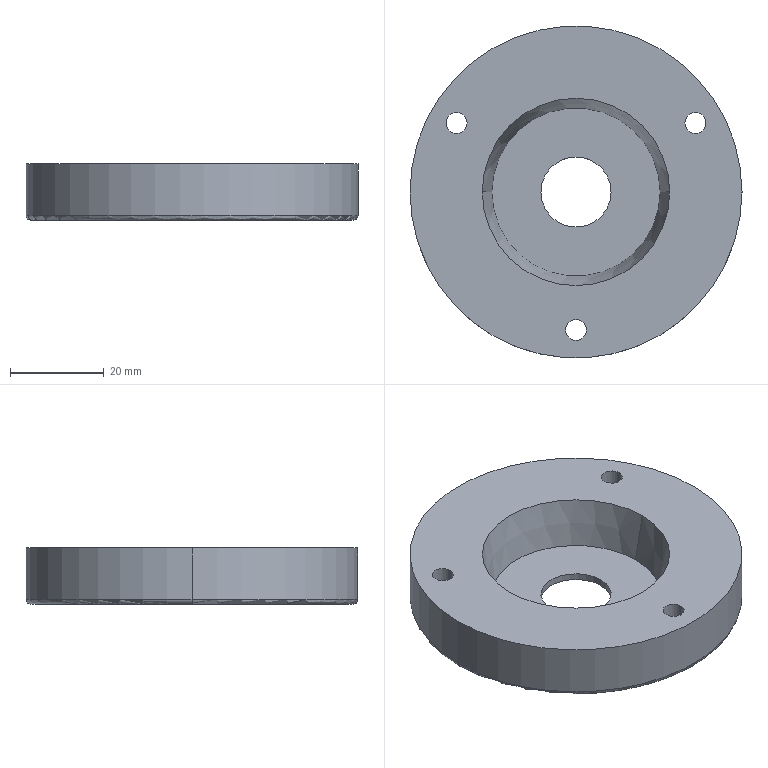Component | SolidWorks | SealingCover-2 | 1 solid | 26 faces | box 71 x 71 x 12 mm | volume 34206 mm3 | cylinder 16 | plane 6 | torus 2 | cone 2 | commonest cylinder face diameters 8 x6 4.5 x6 15 x2 71 x2
build123d program:
from build123d import *

# Parameters (mm, degrees)
SKETCH1_R                                            = 35.5
BOSS_EXTRUDE1_DEPTH                                  = 12
HOLE_SIZE_ACCORDING_TO_HEXAGON_SOCKET_HE_D           = 4.5
HOLE_SIZE_ACCORDING_TO_HEXAGON_SOCKET_HE_CBORE_D     = 8
HOLE_SIZE_ACCORDING_TO_HEXAGON_SOCKET_HE_CBORE_DEPTH = 4.6
CIRPATTERN1_COUNT                                    = 3
FILLET1_R                                            = 1


with BuildPart() as part:
    # Sketch1 → Boss-Extrude1 (new body)
    with BuildSketch(Plane.XY):
        Circle(SKETCH1_R)
    extrude(amount=-BOSS_EXTRUDE1_DEPTH)

    # Sketch2 → Cut-Revolve1 (revolve, cut)
    with BuildSketch(Plane(origin=(0, 0, 0), x_dir=(1, 0, 0), z_dir=(0, 1, 0)), mode=Mode.PRIVATE) as cut_revolve1_sk:
        Polygon((-18, 1.5), (-7.5, 1.5), (-7.5, 0), (0, 0), (0, 12), (-20.041, 12), align=None)
    revolve(cut_revolve1_sk.sketch.rotate(Axis((0, 0, 0), (0, 0, -1)), 180), axis=Axis((0, 0, 0), (0, 0, -1)), mode=Mode.SUBTRACT)

    # Hole Size_According to_Hexagon Socket He (through all)
    with Locations(Plane.XY):
        with Locations((0, -29.5)):
            hole_size_according_to_hexagon_socket_he = CounterBoreHole(HOLE_SIZE_ACCORDING_TO_HEXAGON_SOCKET_HE_D / 2, HOLE_SIZE_ACCORDING_TO_HEXAGON_SOCKET_HE_CBORE_D / 2, HOLE_SIZE_ACCORDING_TO_HEXAGON_SOCKET_HE_CBORE_DEPTH)

    # CirPattern1: Hole Size_According to_Hexagon Socket He ×3 about axis
    cirpattern1_axis = Axis((0, 0, 0), (0, 0, 1))
    for i in range(1, CIRPATTERN1_COUNT):
        add(hole_size_according_to_hexagon_socket_he.rotate(cirpattern1_axis, i * 360 / CIRPATTERN1_COUNT), mode=Mode.SUBTRACT)

    # Fillet1
    fillet1_edges = [part.edges().sort_by_distance(p)[0] for p in [
        (-35.5, 0, 0),
    ]]
    fillet(fillet1_edges, radius=FILLET1_R)


solid = part.part

# Placed as in the assembly
solid = solid.moved(Location((32, 58.948, -59), (-180, 0, 180)))
STEP:
#1=COLOUR_RGB('',0.7922,0.8196,0.9333);
#2=FILL_AREA_STYLE_COLOUR('',#1);
#3=FILL_AREA_STYLE('',(#2));
#4=SURFACE_STYLE_FILL_AREA(#3);
#5=SURFACE_SIDE_STYLE('',(#4));
#6=SURFACE_STYLE_USAGE(.BOTH.,#5);
#7=PRESENTATION_STYLE_ASSIGNMENT((#6));
#8=CARTESIAN_POINT('',(2.657,2.321,-2.283));
#9=VERTEX_POINT('',#8);
#10=CARTESIAN_POINT('',(-0.1378,2.321,-2.283));
#11=VERTEX_POINT('',#10);
#12=CARTESIAN_POINT('',(1.26,2.321,-2.283));
#13=DIRECTION('',(0.,0.,1.));
#14=DIRECTION('',(-1.,-0.,0.));
#15=AXIS2_PLACEMENT_3D('',#12,#13,#14);
#16=CIRCLE('',#15,1.398);
#17=EDGE_CURVE('',#9,#11,#16,.T.);
#18=ORIENTED_EDGE('',*,*,#17,.F.);
#19=CARTESIAN_POINT('',(2.618,2.321,-2.323));
#20=VERTEX_POINT('',#19);
#21=CARTESIAN_POINT('',(2.618,2.321,-2.283));
#22=DIRECTION('',(-0.,1.,-0.));
#23=DIRECTION('',(-1.,0.,0.));
#24=AXIS2_PLACEMENT_3D('',#21,#22,#23);
#25=CIRCLE('',#24,0.03937);
#26=EDGE_CURVE('',#9,#20,#25,.T.);
#27=ORIENTED_EDGE('',*,*,#26,.T.);
#28=CARTESIAN_POINT('',(-0.09843,2.321,-2.323));
#29=VERTEX_POINT('',#28);
#30=CARTESIAN_POINT('',(1.26,2.321,-2.323));
#31=DIRECTION('',(-0.,-0.,-1.));
#32=DIRECTION('',(-1.,-0.,0.));
#33=AXIS2_PLACEMENT_3D('',#30,#31,#32);
#34=CIRCLE('',#33,1.358);
#35=EDGE_CURVE('',#29,#20,#34,.T.);
#36=ORIENTED_EDGE('',*,*,#35,.F.);
#37=CARTESIAN_POINT('',(-0.09843,2.321,-2.283));
#38=DIRECTION('',(0.,-1.,0.));
#39=DIRECTION('',(1.,0.,0.));
#40=AXIS2_PLACEMENT_3D('',#37,#38,#39);
#41=CIRCLE('',#40,0.03937);
#42=EDGE_CURVE('',#11,#29,#41,.T.);
#43=ORIENTED_EDGE('',*,*,#42,.F.);
#44=EDGE_LOOP('',(#18,#27,#36,#43));
#45=FACE_OUTER_BOUND('',#44,.T.);
#46=CARTESIAN_POINT('',(1.26,2.321,-2.283));
#47=DIRECTION('',(-0.,-0.,-1.));
#48=DIRECTION('',(-1.,-0.,0.));
#49=AXIS2_PLACEMENT_3D('',#46,#47,#48);
#50=TOROIDAL_SURFACE('',#49,1.358,0.03937);
#51=ADVANCED_FACE('',(#45),#50,.T.);
#52=CARTESIAN_POINT('',(0.4115,2.901,-2.142));
#53=VERTEX_POINT('',#52);
#54=CARTESIAN_POINT('',(0.09655,2.901,-2.142));
#55=VERTEX_POINT('',#54);
#56=CARTESIAN_POINT('',(0.254,2.901,-2.142));
#57=DIRECTION('',(-0.,-0.,-1.));
#58=DIRECTION('',(-1.,0.,0.));
#59=AXIS2_PLACEMENT_3D('',#56,#57,#58);
#60=CIRCLE('',#59,0.1575);
#61=EDGE_CURVE('',#53,#55,#60,.T.);
#62=ORIENTED_EDGE('',*,*,#61,.F.);
#63=CARTESIAN_POINT('',(0.4115,2.901,-2.323));
#64=VERTEX_POINT('',#63);
#65=CARTESIAN_POINT('',(0.4115,2.901,-2.323));
#66=DIRECTION('',(-0.,-0.,-1.));
#67=VECTOR('',#66,39.37);
#68=LINE('',#65,#67);
#69=EDGE_CURVE('',#53,#64,#68,.T.);
#70=ORIENTED_EDGE('',*,*,#69,.T.);
#71=CARTESIAN_POINT('',(0.09655,2.901,-2.323));
#72=VERTEX_POINT('',#71);
#73=CARTESIAN_POINT('',(0.254,2.901,-2.323));
#74=DIRECTION('',(-0.,-0.,-1.));
#75=DIRECTION('',(-1.,0.,0.));
#76=AXIS2_PLACEMENT_3D('',#73,#74,#75);
#77=CIRCLE('',#76,0.1575);
#78=EDGE_CURVE('',#64,#72,#77,.T.);
#79=ORIENTED_EDGE('',*,*,#78,.T.);
#80=CARTESIAN_POINT('',(0.09655,2.901,-2.323));
#81=DIRECTION('',(-0.,-0.,-1.));
#82=VECTOR('',#81,39.37);
#83=LINE('',#80,#82);
#84=EDGE_CURVE('',#55,#72,#83,.T.);
#85=ORIENTED_EDGE('',*,*,#84,.F.);
#86=EDGE_LOOP('',(#62,#70,#79,#85));
#87=FACE_OUTER_BOUND('',#86,.T.);
#88=CARTESIAN_POINT('',(0.254,2.901,-2.323));
#89=DIRECTION('',(-0.,-0.,-1.));
#90=DIRECTION('',(-1.,0.,0.));
#91=AXIS2_PLACEMENT_3D('',#88,#89,#90);
#92=CYLINDRICAL_SURFACE('',#91,0.1575);
#93=ADVANCED_FACE('',(#87),#92,.F.);
#94=CARTESIAN_POINT('',(0.3426,2.901,-1.85));
#95=VERTEX_POINT('',#94);
#96=CARTESIAN_POINT('',(0.1654,2.901,-1.85));
#97=VERTEX_POINT('',#96);
#98=CARTESIAN_POINT('',(0.254,2.901,-1.85));
#99=DIRECTION('',(-0.,-0.,-1.));
#100=DIRECTION('',(-1.,0.,0.));
#101=AXIS2_PLACEMENT_3D('',#98,#99,#100);
#102=CIRCLE('',#101,0.08858);
#103=EDGE_CURVE('',#95,#97,#102,.T.);
#104=ORIENTED_EDGE('',*,*,#103,.F.);
#105=CARTESIAN_POINT('',(0.3426,2.901,-2.142));
#106=VERTEX_POINT('',#105);
#107=CARTESIAN_POINT('',(0.3426,2.901,-2.323));
#108=DIRECTION('',(-0.,-0.,-1.));
#109=VECTOR('',#108,39.37);
#110=LINE('',#107,#109);
#111=EDGE_CURVE('',#95,#106,#110,.T.);
#112=ORIENTED_EDGE('',*,*,#111,.T.);
#113=CARTESIAN_POINT('',(0.1654,2.901,-2.142));
#114=VERTEX_POINT('',#113);
#115=CARTESIAN_POINT('',(0.254,2.901,-2.142));
#116=DIRECTION('',(-0.,-0.,-1.));
#117=DIRECTION('',(-1.,0.,0.));
#118=AXIS2_PLACEMENT_3D('',#115,#116,#117);
#119=CIRCLE('',#118,0.08858);
#120=EDGE_CURVE('',#106,#114,#119,.T.);
#121=ORIENTED_EDGE('',*,*,#120,.T.);
#122=CARTESIAN_POINT('',(0.1654,2.901,-2.323));
#123=DIRECTION('',(-0.,-0.,-1.));
#124=VECTOR('',#123,39.37);
#125=LINE('',#122,#124);
#126=EDGE_CURVE('',#97,#114,#125,.T.);
#127=ORIENTED_EDGE('',*,*,#126,.F.);
#128=EDGE_LOOP('',(#104,#112,#121,#127));
#129=FACE_OUTER_BOUND('',#128,.T.);
#130=CARTESIAN_POINT('',(0.254,2.901,-2.323));
#131=DIRECTION('',(-0.,-0.,-1.));
#132=DIRECTION('',(-1.,0.,0.));
#133=AXIS2_PLACEMENT_3D('',#130,#131,#132);
#134=CYLINDRICAL_SURFACE('',#133,0.08858);
#135=ADVANCED_FACE('',(#129),#134,.F.);
#136=CARTESIAN_POINT('',(2.423,2.901,-2.142));
#137=VERTEX_POINT('',#136);
#138=CARTESIAN_POINT('',(2.108,2.901,-2.142));
#139=VERTEX_POINT('',#138);
#140=CARTESIAN_POINT('',(2.266,2.901,-2.142));
#141=DIRECTION('',(-0.,-0.,-1.));
#142=DIRECTION('',(-1.,0.,0.));
#143=AXIS2_PLACEMENT_3D('',#140,#141,#142);
#144=CIRCLE('',#143,0.1575);
#145=EDGE_CURVE('',#137,#139,#144,.T.);
#146=ORIENTED_EDGE('',*,*,#145,.F.);
#147=CARTESIAN_POINT('',(2.423,2.901,-2.323));
#148=VERTEX_POINT('',#147);
#149=CARTESIAN_POINT('',(2.423,2.901,-2.323));
#150=DIRECTION('',(-0.,-0.,-1.));
#151=VECTOR('',#150,39.37);
#152=LINE('',#149,#151);
#153=EDGE_CURVE('',#137,#148,#152,.T.);
#154=ORIENTED_EDGE('',*,*,#153,.T.);
#155=CARTESIAN_POINT('',(2.108,2.901,-2.323));
#156=VERTEX_POINT('',#155);
#157=CARTESIAN_POINT('',(2.266,2.901,-2.323));
#158=DIRECTION('',(-0.,-0.,-1.));
#159=DIRECTION('',(-1.,0.,0.));
#160=AXIS2_PLACEMENT_3D('',#157,#158,#159);
#161=CIRCLE('',#160,0.1575);
#162=EDGE_CURVE('',#148,#156,#161,.T.);
#163=ORIENTED_EDGE('',*,*,#162,.T.);
#164=CARTESIAN_POINT('',(2.108,2.901,-2.323));
#165=DIRECTION('',(-0.,-0.,-1.));
#166=VECTOR('',#165,39.37);
#167=LINE('',#164,#166);
#168=EDGE_CURVE('',#139,#156,#167,.T.);
#169=ORIENTED_EDGE('',*,*,#168,.F.);
#170=EDGE_LOOP('',(#146,#154,#163,#169));
#171=FACE_OUTER_BOUND('',#170,.T.);
#172=CARTESIAN_POINT('',(2.266,2.901,-2.323));
#173=DIRECTION('',(-0.,-0.,-1.));
#174=DIRECTION('',(-1.,0.,0.));
#175=AXIS2_PLACEMENT_3D('',#172,#173,#174);
#176=CYLINDRICAL_SURFACE('',#175,0.1575);
#177=ADVANCED_FACE('',(#171),#176,.F.);
#178=CARTESIAN_POINT('',(2.354,2.901,-1.85));
#179=VERTEX_POINT('',#178);
#180=CARTESIAN_POINT('',(2.177,2.901,-1.85));
#181=VERTEX_POINT('',#180);
#182=CARTESIAN_POINT('',(2.266,2.901,-1.85));
#183=DIRECTION('',(-0.,-0.,-1.));
#184=DIRECTION('',(-1.,0.,0.));
#185=AXIS2_PLACEMENT_3D('',#182,#183,#184);
#186=CIRCLE('',#185,0.08858);
#187=EDGE_CURVE('',#179,#181,#186,.T.);
#188=ORIENTED_EDGE('',*,*,#187,.F.);
#189=CARTESIAN_POINT('',(2.354,2.901,-2.142));
#190=VERTEX_POINT('',#189);
#191=CARTESIAN_POINT('',(2.354,2.901,-2.323));
#192=DIRECTION('',(-0.,-0.,-1.));
#193=VECTOR('',#192,39.37);
#194=LINE('',#191,#193);
#195=EDGE_CURVE('',#179,#190,#194,.T.);
#196=ORIENTED_EDGE('',*,*,#195,.T.);
#197=CARTESIAN_POINT('',(2.177,2.901,-2.142));
#198=VERTEX_POINT('',#197);
#199=CARTESIAN_POINT('',(2.266,2.901,-2.142));
#200=DIRECTION('',(-0.,-0.,-1.));
#201=DIRECTION('',(-1.,0.,0.));
#202=AXIS2_PLACEMENT_3D('',#199,#200,#201);
#203=CIRCLE('',#202,0.08858);
#204=EDGE_CURVE('',#190,#198,#203,.T.);
#205=ORIENTED_EDGE('',*,*,#204,.T.);
#206=CARTESIAN_POINT('',(2.177,2.901,-2.323));
#207=DIRECTION('',(-0.,-0.,-1.));
#208=VECTOR('',#207,39.37);
#209=LINE('',#206,#208);
#210=EDGE_CURVE('',#181,#198,#209,.T.);
#211=ORIENTED_EDGE('',*,*,#210,.F.);
#212=EDGE_LOOP('',(#188,#196,#205,#211));
#213=FACE_OUTER_BOUND('',#212,.T.);
#214=CARTESIAN_POINT('',(2.266,2.901,-2.323));
#215=DIRECTION('',(-0.,-0.,-1.));
#216=DIRECTION('',(-1.,0.,0.));
#217=AXIS2_PLACEMENT_3D('',#214,#215,#216);
#218=CYLINDRICAL_SURFACE('',#217,0.08858);
#219=ADVANCED_FACE('',(#213),#218,.F.);
#220=CARTESIAN_POINT('',(1.417,1.159,-2.142));
#221=VERTEX_POINT('',#220);
#222=CARTESIAN_POINT('',(1.102,1.159,-2.142));
#223=VERTEX_POINT('',#222);
#224=CARTESIAN_POINT('',(1.26,1.159,-2.142));
#225=DIRECTION('',(-0.,-0.,-1.));
#226=DIRECTION('',(-1.,-0.,0.));
#227=AXIS2_PLACEMENT_3D('',#224,#225,#226);
#228=CIRCLE('',#227,0.1575);
#229=EDGE_CURVE('',#221,#223,#228,.T.);
#230=ORIENTED_EDGE('',*,*,#229,.F.);
#231=CARTESIAN_POINT('',(1.417,1.159,-2.323));
#232=VERTEX_POINT('',#231);
#233=CARTESIAN_POINT('',(1.417,1.159,-2.323));
#234=DIRECTION('',(-0.,-0.,-1.));
#235=VECTOR('',#234,39.37);
#236=LINE('',#233,#235);
#237=EDGE_CURVE('',#221,#232,#236,.T.);
#238=ORIENTED_EDGE('',*,*,#237,.T.);
#239=CARTESIAN_POINT('',(1.102,1.159,-2.323));
#240=VERTEX_POINT('',#239);
#241=CARTESIAN_POINT('',(1.26,1.159,-2.323));
#242=DIRECTION('',(-0.,-0.,-1.));
#243=DIRECTION('',(-1.,-0.,0.));
#244=AXIS2_PLACEMENT_3D('',#241,#242,#243);
#245=CIRCLE('',#244,0.1575);
#246=EDGE_CURVE('',#232,#240,#245,.T.);
#247=ORIENTED_EDGE('',*,*,#246,.T.);
#248=CARTESIAN_POINT('',(1.102,1.159,-2.323));
#249=DIRECTION('',(-0.,-0.,-1.));
#250=VECTOR('',#249,39.37);
#251=LINE('',#248,#250);
#252=EDGE_CURVE('',#223,#240,#251,.T.);
#253=ORIENTED_EDGE('',*,*,#252,.F.);
#254=EDGE_LOOP('',(#230,#238,#247,#253));
#255=FACE_OUTER_BOUND('',#254,.T.);
#256=CARTESIAN_POINT('',(1.26,1.159,-2.323));
#257=DIRECTION('',(-0.,-0.,-1.));
#258=DIRECTION('',(-1.,-0.,0.));
#259=AXIS2_PLACEMENT_3D('',#256,#257,#258);
#260=CYLINDRICAL_SURFACE('',#259,0.1575);
#261=ADVANCED_FACE('',(#255),#260,.F.);
#262=CARTESIAN_POINT('',(1.348,1.159,-1.85));
#263=VERTEX_POINT('',#262);
#264=CARTESIAN_POINT('',(1.171,1.159,-1.85));
#265=VERTEX_POINT('',#264);
#266=CARTESIAN_POINT('',(1.26,1.159,-1.85));
#267=DIRECTION('',(-0.,-0.,-1.));
#268=DIRECTION('',(-1.,-0.,0.));
#269=AXIS2_PLACEMENT_3D('',#266,#267,#268);
#270=CIRCLE('',#269,0.08858);
#271=EDGE_CURVE('',#263,#265,#270,.T.);
#272=ORIENTED_EDGE('',*,*,#271,.F.);
#273=CARTESIAN_POINT('',(1.348,1.159,-2.142));
#274=VERTEX_POINT('',#273);
#275=CARTESIAN_POINT('',(1.348,1.159,-2.323));
#276=DIRECTION('',(-0.,-0.,-1.));
#277=VECTOR('',#276,39.37);
#278=LINE('',#275,#277);
#279=EDGE_CURVE('',#263,#274,#278,.T.);
#280=ORIENTED_EDGE('',*,*,#279,.T.);
#281=CARTESIAN_POINT('',(1.171,1.159,-2.142));
#282=VERTEX_POINT('',#281);
#283=CARTESIAN_POINT('',(1.26,1.159,-2.142));
#284=DIRECTION('',(-0.,-0.,-1.));
#285=DIRECTION('',(-1.,-0.,0.));
#286=AXIS2_PLACEMENT_3D('',#283,#284,#285);
#287=CIRCLE('',#286,0.08858);
#288=EDGE_CURVE('',#274,#282,#287,.T.);
#289=ORIENTED_EDGE('',*,*,#288,.T.);
#290=CARTESIAN_POINT('',(1.171,1.159,-2.323));
#291=DIRECTION('',(-0.,-0.,-1.));
#292=VECTOR('',#291,39.37);
#293=LINE('',#290,#292);
#294=EDGE_CURVE('',#265,#282,#293,.T.);
#295=ORIENTED_EDGE('',*,*,#294,.F.);
#296=EDGE_LOOP('',(#272,#280,#289,#295));
#297=FACE_OUTER_BOUND('',#296,.T.);
#298=CARTESIAN_POINT('',(1.26,1.159,-2.323));
#299=DIRECTION('',(-0.,-0.,-1.));
#300=DIRECTION('',(-1.,-0.,0.));
#301=AXIS2_PLACEMENT_3D('',#298,#299,#300);
#302=CYLINDRICAL_SURFACE('',#301,0.08858);
#303=ADVANCED_FACE('',(#297),#302,.F.);
#304=CARTESIAN_POINT('',(1.555,2.321,-2.264));
#305=VERTEX_POINT('',#304);
#306=CARTESIAN_POINT('',(0.9646,2.321,-2.264));
#307=VERTEX_POINT('',#306);
#308=CARTESIAN_POINT('',(1.26,2.321,-2.264));
#309=DIRECTION('',(-0.,-0.,-1.));
#310=DIRECTION('',(-1.,-0.,0.));
#311=AXIS2_PLACEMENT_3D('',#308,#309,#310);
#312=CIRCLE('',#311,0.2953);
#313=EDGE_CURVE('',#305,#307,#312,.T.);
#314=ORIENTED_EDGE('',*,*,#313,.F.);
#315=CARTESIAN_POINT('',(1.555,2.321,-2.323));
#316=VERTEX_POINT('',#315);
#317=CARTESIAN_POINT('',(1.555,2.321,-2.323));
#318=DIRECTION('',(-0.,-0.,-1.));
#319=VECTOR('',#318,39.37);
#320=LINE('',#317,#319);
#321=EDGE_CURVE('',#305,#316,#320,.T.);
#322=ORIENTED_EDGE('',*,*,#321,.T.);
#323=CARTESIAN_POINT('',(0.9646,2.321,-2.323));
#324=VERTEX_POINT('',#323);
#325=CARTESIAN_POINT('',(1.26,2.321,-2.323));
#326=DIRECTION('',(-0.,-0.,-1.));
#327=DIRECTION('',(-1.,-0.,0.));
#328=AXIS2_PLACEMENT_3D('',#325,#326,#327);
#329=CIRCLE('',#328,0.2953);
#330=EDGE_CURVE('',#316,#324,#329,.T.);
#331=ORIENTED_EDGE('',*,*,#330,.T.);
#332=CARTESIAN_POINT('',(0.9646,2.321,-2.323));
#333=DIRECTION('',(-0.,-0.,-1.));
#334=VECTOR('',#333,39.37);
#335=LINE('',#332,#334);
#336=EDGE_CURVE('',#307,#324,#335,.T.);
#337=ORIENTED_EDGE('',*,*,#336,.F.);
#338=EDGE_LOOP('',(#314,#322,#331,#337));
#339=FACE_OUTER_BOUND('',#338,.T.);
#340=CARTESIAN_POINT('',(1.26,2.321,-2.323));
#341=DIRECTION('',(-0.,-0.,-1.));
#342=DIRECTION('',(-1.,-0.,0.));
#343=AXIS2_PLACEMENT_3D('',#340,#341,#342);
#344=CYLINDRICAL_SURFACE('',#343,0.2953);
#345=ADVANCED_FACE('',(#339),#344,.F.);
#346=CARTESIAN_POINT('',(1.969,2.321,-2.264));
#347=VERTEX_POINT('',#346);
#348=CARTESIAN_POINT('',(0.5512,2.321,-2.264));
#349=VERTEX_POINT('',#348);
#350=CARTESIAN_POINT('',(1.26,2.321,-2.264));
#351=DIRECTION('',(-0.,-0.,-1.));
#352=DIRECTION('',(-1.,-0.,0.));
#353=AXIS2_PLACEMENT_3D('',#350,#351,#352);
#354=CIRCLE('',#353,0.7087);
#355=EDGE_CURVE('',#347,#349,#354,.T.);
#356=ORIENTED_EDGE('',*,*,#355,.T.);
#357=CARTESIAN_POINT('',(0.4708,2.321,-1.85));
#358=VERTEX_POINT('',#357);
#359=CARTESIAN_POINT('',(0.4708,2.321,-1.85));
#360=DIRECTION('',(-0.1908,0.,0.9816));
#361=VECTOR('',#360,39.37);
#362=LINE('',#359,#361);
#363=EDGE_CURVE('',#349,#358,#362,.T.);
#364=ORIENTED_EDGE('',*,*,#363,.T.);
#365=CARTESIAN_POINT('',(2.049,2.321,-1.85));
#366=VERTEX_POINT('',#365);
#367=CARTESIAN_POINT('',(1.26,2.321,-1.85));
#368=DIRECTION('',(-0.,-0.,-1.));
#369=DIRECTION('',(-1.,-0.,0.));
#370=AXIS2_PLACEMENT_3D('',#367,#368,#369);
#371=CIRCLE('',#370,0.789);
#372=EDGE_CURVE('',#366,#358,#371,.T.);
#373=ORIENTED_EDGE('',*,*,#372,.F.);
#374=CARTESIAN_POINT('',(2.049,2.321,-1.85));
#375=DIRECTION('',(0.1908,0.,0.9816));
#376=VECTOR('',#375,39.37);
#377=LINE('',#374,#376);
#378=EDGE_CURVE('',#347,#366,#377,.T.);
#379=ORIENTED_EDGE('',*,*,#378,.F.);
#380=EDGE_LOOP('',(#356,#364,#373,#379));
#381=FACE_OUTER_BOUND('',#380,.T.);
#382=CARTESIAN_POINT('',(1.26,2.321,-1.85));
#383=DIRECTION('',(0.,0.,1.));
#384=DIRECTION('',(1.,0.,0.));
#385=AXIS2_PLACEMENT_3D('',#382,#383,#384);
#386=CONICAL_SURFACE('',#385,0.789,0.192);
#387=ADVANCED_FACE('',(#381),#386,.F.);
#388=CARTESIAN_POINT('',(-0.1378,2.321,-1.85));
#389=VERTEX_POINT('',#388);
#390=CARTESIAN_POINT('',(2.657,2.321,-1.85));
#391=VERTEX_POINT('',#390);
#392=CARTESIAN_POINT('',(1.26,2.321,-1.85));
#393=DIRECTION('',(-0.,-0.,-1.));
#394=DIRECTION('',(-1.,-0.,0.));
#395=AXIS2_PLACEMENT_3D('',#392,#393,#394);
#396=CIRCLE('',#395,1.398);
#397=EDGE_CURVE('',#389,#391,#396,.T.);
#398=ORIENTED_EDGE('',*,*,#397,.T.);
#399=CARTESIAN_POINT('',(2.657,2.321,-1.85));
#400=DIRECTION('',(-0.,-0.,-1.));
#401=VECTOR('',#400,39.37);
#402=LINE('',#399,#401);
#403=EDGE_CURVE('',#391,#9,#402,.T.);
#404=ORIENTED_EDGE('',*,*,#403,.T.);
#405=ORIENTED_EDGE('',*,*,#17,.T.);
#406=CARTESIAN_POINT('',(-0.1378,2.321,-1.85));
#407=DIRECTION('',(-0.,-0.,-1.));
#408=VECTOR('',#407,39.37);
#409=LINE('',#406,#408);
#410=EDGE_CURVE('',#389,#11,#409,.T.);
#411=ORIENTED_EDGE('',*,*,#410,.F.);
#412=EDGE_LOOP('',(#398,#404,#405,#411));
#413=FACE_OUTER_BOUND('',#412,.T.);
#414=CARTESIAN_POINT('',(1.26,2.321,-1.85));
#415=DIRECTION('',(-0.,-0.,-1.));
#416=DIRECTION('',(-1.,-0.,0.));
#417=AXIS2_PLACEMENT_3D('',#414,#415,#416);
#418=CYLINDRICAL_SURFACE('',#417,1.398);
#419=ADVANCED_FACE('',(#413),#418,.T.);
#420=ORIENTED_EDGE('',*,*,#403,.F.);
#421=CARTESIAN_POINT('',(1.26,2.321,-1.85));
#422=DIRECTION('',(-0.,-0.,-1.));
#423=DIRECTION('',(-1.,-0.,0.));
#424=AXIS2_PLACEMENT_3D('',#421,#422,#423);
#425=CIRCLE('',#424,1.398);
#426=EDGE_CURVE('',#391,#389,#425,.T.);
#427=ORIENTED_EDGE('',*,*,#426,.T.);
#428=ORIENTED_EDGE('',*,*,#410,.T.);
#429=CARTESIAN_POINT('',(1.26,2.321,-2.283));
#430=DIRECTION('',(0.,0.,1.));
#431=DIRECTION('',(-1.,-0.,0.));
#432=AXIS2_PLACEMENT_3D('',#429,#430,#431);
#433=CIRCLE('',#432,1.398);
#434=EDGE_CURVE('',#11,#9,#433,.T.);
#435=ORIENTED_EDGE('',*,*,#434,.T.);
#436=EDGE_LOOP('',(#420,#427,#428,#435));
#437=FACE_OUTER_BOUND('',#436,.T.);
#438=CARTESIAN_POINT('',(1.26,2.321,-1.85));
#439=DIRECTION('',(-0.,-0.,-1.));
#440=DIRECTION('',(-1.,-0.,0.));
#441=AXIS2_PLACEMENT_3D('',#438,#439,#440);
#442=CYLINDRICAL_SURFACE('',#441,1.398);
#443=ADVANCED_FACE('',(#437),#442,.T.);
#444=CARTESIAN_POINT('',(0.254,2.901,-1.85));
#445=DIRECTION('',(-0.,-0.,-1.));
#446=DIRECTION('',(-1.,0.,0.));
#447=AXIS2_PLACEMENT_3D('',#444,#445,#446);
#448=CIRCLE('',#447,0.08858);
#449=EDGE_CURVE('',#97,#95,#448,.T.);
#450=ORIENTED_EDGE('',*,*,#449,.T.);
#451=ORIENTED_EDGE('',*,*,#103,.T.);
#452=EDGE_LOOP('',(#450,#451));
#453=FACE_BOUND('',#452,.T.);
#454=CARTESIAN_POINT('',(2.266,2.901,-1.85));
#455=DIRECTION('',(-0.,-0.,-1.));
#456=DIRECTION('',(-1.,0.,0.));
#457=AXIS2_PLACEMENT_3D('',#454,#455,#456);
#458=CIRCLE('',#457,0.08858);
#459=EDGE_CURVE('',#181,#179,#458,.T.);
#460=ORIENTED_EDGE('',*,*,#459,.T.);
#461=ORIENTED_EDGE('',*,*,#187,.T.);
#462=EDGE_LOOP('',(#460,#461));
#463=FACE_BOUND('',#462,.T.);
#464=CARTESIAN_POINT('',(1.26,1.159,-1.85));
#465=DIRECTION('',(-0.,-0.,-1.));
#466=DIRECTION('',(-1.,-0.,0.));
#467=AXIS2_PLACEMENT_3D('',#464,#465,#466);
#468=CIRCLE('',#467,0.08858);
#469=EDGE_CURVE('',#265,#263,#468,.T.);
#470=ORIENTED_EDGE('',*,*,#469,.T.);
#471=ORIENTED_EDGE('',*,*,#271,.T.);
#472=EDGE_LOOP('',(#470,#471));
#473=FACE_BOUND('',#472,.T.);
#474=ORIENTED_EDGE('',*,*,#372,.T.);
#475=CARTESIAN_POINT('',(1.26,2.321,-1.85));
#476=DIRECTION('',(-0.,-0.,-1.));
#477=DIRECTION('',(-1.,-0.,0.));
#478=AXIS2_PLACEMENT_3D('',#475,#476,#477);
#479=CIRCLE('',#478,0.789);
#480=EDGE_CURVE('',#358,#366,#479,.T.);
#481=ORIENTED_EDGE('',*,*,#480,.T.);
#482=EDGE_LOOP('',(#474,#481));
#483=FACE_BOUND('',#482,.T.);
#484=ORIENTED_EDGE('',*,*,#397,.F.);
#485=ORIENTED_EDGE('',*,*,#426,.F.);
#486=EDGE_LOOP('',(#484,#485));
#487=FACE_OUTER_BOUND('',#486,.T.);
#488=CARTESIAN_POINT('',(1.26,2.321,-1.85));
#489=DIRECTION('',(-0.,-0.,-1.));
#490=DIRECTION('',(-1.,-0.,0.));
#491=AXIS2_PLACEMENT_3D('',#488,#489,#490);
#492=PLANE('',#491);
#493=ADVANCED_FACE('',(#453,#463,#473,#483,#487),#492,.F.);
#494=ORIENTED_EDGE('',*,*,#35,.T.);
#495=CARTESIAN_POINT('',(1.26,2.321,-2.323));
#496=DIRECTION('',(-0.,-0.,-1.));
#497=DIRECTION('',(-1.,-0.,0.));
#498=AXIS2_PLACEMENT_3D('',#495,#496,#497);
#499=CIRCLE('',#498,1.358);
#500=EDGE_CURVE('',#20,#29,#499,.T.);
#501=ORIENTED_EDGE('',*,*,#500,.T.);
#502=EDGE_LOOP('',(#494,#501));
#503=FACE_OUTER_BOUND('',#502,.T.);
#504=CARTESIAN_POINT('',(0.254,2.901,-2.323));
#505=DIRECTION('',(-0.,-0.,-1.));
#506=DIRECTION('',(-1.,0.,0.));
#507=AXIS2_PLACEMENT_3D('',#504,#505,#506);
#508=CIRCLE('',#507,0.1575);
#509=EDGE_CURVE('',#72,#64,#508,.T.);
#510=ORIENTED_EDGE('',*,*,#509,.F.);
#511=ORIENTED_EDGE('',*,*,#78,.F.);
#512=EDGE_LOOP('',(#510,#511));
#513=FACE_BOUND('',#512,.T.);
#514=CARTESIAN_POINT('',(2.266,2.901,-2.323));
#515=DIRECTION('',(-0.,-0.,-1.));
#516=DIRECTION('',(-1.,0.,0.));
#517=AXIS2_PLACEMENT_3D('',#514,#515,#516);
#518=CIRCLE('',#517,0.1575);
#519=EDGE_CURVE('',#156,#148,#518,.T.);
#520=ORIENTED_EDGE('',*,*,#519,.F.);
#521=ORIENTED_EDGE('',*,*,#162,.F.);
#522=EDGE_LOOP('',(#520,#521));
#523=FACE_BOUND('',#522,.T.);
#524=CARTESIAN_POINT('',(1.26,1.159,-2.323));
#525=DIRECTION('',(-0.,-0.,-1.));
#526=DIRECTION('',(-1.,-0.,0.));
#527=AXIS2_PLACEMENT_3D('',#524,#525,#526);
#528=CIRCLE('',#527,0.1575);
#529=EDGE_CURVE('',#240,#232,#528,.T.);
#530=ORIENTED_EDGE('',*,*,#529,.F.);
#531=ORIENTED_EDGE('',*,*,#246,.F.);
#532=EDGE_LOOP('',(#530,#531));
#533=FACE_BOUND('',#532,.T.);
#534=CARTESIAN_POINT('',(1.26,2.321,-2.323));
#535=DIRECTION('',(-0.,-0.,-1.));
#536=DIRECTION('',(-1.,-0.,0.));
#537=AXIS2_PLACEMENT_3D('',#534,#535,#536);
#538=CIRCLE('',#537,0.2953);
#539=EDGE_CURVE('',#324,#316,#538,.T.);
#540=ORIENTED_EDGE('',*,*,#539,.F.);
#541=ORIENTED_EDGE('',*,*,#330,.F.);
#542=EDGE_LOOP('',(#540,#541));
#543=FACE_BOUND('',#542,.T.);
#544=CARTESIAN_POINT('',(1.26,2.321,-2.323));
#545=DIRECTION('',(-0.,-0.,-1.));
#546=DIRECTION('',(-1.,-0.,0.));
#547=AXIS2_PLACEMENT_3D('',#544,#545,#546);
#548=PLANE('',#547);
#549=ADVANCED_FACE('',(#503,#513,#523,#533,#543),#548,.T.);
#550=ORIENTED_EDGE('',*,*,#363,.F.);
#551=CARTESIAN_POINT('',(1.26,2.321,-2.264));
#552=DIRECTION('',(-0.,-0.,-1.));
#553=DIRECTION('',(-1.,-0.,0.));
#554=AXIS2_PLACEMENT_3D('',#551,#552,#553);
#555=CIRCLE('',#554,0.7087);
#556=EDGE_CURVE('',#349,#347,#555,.T.);
#557=ORIENTED_EDGE('',*,*,#556,.T.);
#558=ORIENTED_EDGE('',*,*,#378,.T.);
#559=ORIENTED_EDGE('',*,*,#480,.F.);
#560=EDGE_LOOP('',(#550,#557,#558,#559));
#561=FACE_OUTER_BOUND('',#560,.T.);
#562=CARTESIAN_POINT('',(1.26,2.321,-1.85));
#563=DIRECTION('',(0.,0.,1.));
#564=DIRECTION('',(1.,0.,0.));
#565=AXIS2_PLACEMENT_3D('',#562,#563,#564);
#566=CONICAL_SURFACE('',#565,0.789,0.192);
#567=ADVANCED_FACE('',(#561),#566,.F.);
#568=CARTESIAN_POINT('',(1.26,2.321,-2.264));
#569=DIRECTION('',(-0.,-0.,-1.));
#570=DIRECTION('',(-1.,-0.,0.));
#571=AXIS2_PLACEMENT_3D('',#568,#569,#570);
#572=CIRCLE('',#571,0.2953);
#573=EDGE_CURVE('',#307,#305,#572,.T.);
#574=ORIENTED_EDGE('',*,*,#573,.T.);
#575=ORIENTED_EDGE('',*,*,#313,.T.);
#576=EDGE_LOOP('',(#574,#575));
#577=FACE_BOUND('',#576,.T.);
#578=ORIENTED_EDGE('',*,*,#355,.F.);
#579=ORIENTED_EDGE('',*,*,#556,.F.);
#580=EDGE_LOOP('',(#578,#579));
#581=FACE_OUTER_BOUND('',#580,.T.);
#582=CARTESIAN_POINT('',(1.969,2.321,-2.264));
#583=DIRECTION('',(0.,0.,1.));
#584=DIRECTION('',(1.,0.,-0.));
#585=AXIS2_PLACEMENT_3D('',#582,#583,#584);
#586=PLANE('',#585);
#587=ADVANCED_FACE('',(#577,#581),#586,.T.);
#588=ORIENTED_EDGE('',*,*,#321,.F.);
#589=ORIENTED_EDGE('',*,*,#573,.F.);
#590=ORIENTED_EDGE('',*,*,#336,.T.);
#591=ORIENTED_EDGE('',*,*,#539,.T.);
#592=EDGE_LOOP('',(#588,#589,#590,#591));
#593=FACE_OUTER_BOUND('',#592,.T.);
#594=CARTESIAN_POINT('',(1.26,2.321,-2.323));
#595=DIRECTION('',(-0.,-0.,-1.));
#596=DIRECTION('',(-1.,-0.,0.));
#597=AXIS2_PLACEMENT_3D('',#594,#595,#596);
#598=CYLINDRICAL_SURFACE('',#597,0.2953);
#599=ADVANCED_FACE('',(#593),#598,.F.);
#600=ORIENTED_EDGE('',*,*,#279,.F.);
#601=ORIENTED_EDGE('',*,*,#469,.F.);
#602=ORIENTED_EDGE('',*,*,#294,.T.);
#603=CARTESIAN_POINT('',(1.26,1.159,-2.142));
#604=DIRECTION('',(-0.,-0.,-1.));
#605=DIRECTION('',(-1.,-0.,0.));
#606=AXIS2_PLACEMENT_3D('',#603,#604,#605);
#607=CIRCLE('',#606,0.08858);
#608=EDGE_CURVE('',#282,#274,#607,.T.);
#609=ORIENTED_EDGE('',*,*,#608,.T.);
#610=EDGE_LOOP('',(#600,#601,#602,#609));
#611=FACE_OUTER_BOUND('',#610,.T.);
#612=CARTESIAN_POINT('',(1.26,1.159,-2.323));
#613=DIRECTION('',(-0.,-0.,-1.));
#614=DIRECTION('',(-1.,-0.,0.));
#615=AXIS2_PLACEMENT_3D('',#612,#613,#614);
#616=CYLINDRICAL_SURFACE('',#615,0.08858);
#617=ADVANCED_FACE('',(#611),#616,.F.);
#618=ORIENTED_EDGE('',*,*,#608,.F.);
#619=ORIENTED_EDGE('',*,*,#288,.F.);
#620=EDGE_LOOP('',(#618,#619));
#621=FACE_BOUND('',#620,.T.);
#622=CARTESIAN_POINT('',(1.26,1.159,-2.142));
#623=DIRECTION('',(-0.,-0.,-1.));
#624=DIRECTION('',(-1.,-0.,0.));
#625=AXIS2_PLACEMENT_3D('',#622,#623,#624);
#626=CIRCLE('',#625,0.1575);
#627=EDGE_CURVE('',#223,#221,#626,.T.);
#628=ORIENTED_EDGE('',*,*,#627,.T.);
#629=ORIENTED_EDGE('',*,*,#229,.T.);
#630=EDGE_LOOP('',(#628,#629));
#631=FACE_OUTER_BOUND('',#630,.T.);
#632=CARTESIAN_POINT('',(1.171,1.159,-2.142));
#633=DIRECTION('',(0.,0.,1.));
#634=DIRECTION('',(1.,0.,-0.));
#635=AXIS2_PLACEMENT_3D('',#632,#633,#634);
#636=PLANE('',#635);
#637=ADVANCED_FACE('',(#621,#631),#636,.F.);
#638=ORIENTED_EDGE('',*,*,#237,.F.);
#639=ORIENTED_EDGE('',*,*,#627,.F.);
#640=ORIENTED_EDGE('',*,*,#252,.T.);
#641=ORIENTED_EDGE('',*,*,#529,.T.);
#642=EDGE_LOOP('',(#638,#639,#640,#641));
#643=FACE_OUTER_BOUND('',#642,.T.);
#644=CARTESIAN_POINT('',(1.26,1.159,-2.323));
#645=DIRECTION('',(-0.,-0.,-1.));
#646=DIRECTION('',(-1.,-0.,0.));
#647=AXIS2_PLACEMENT_3D('',#644,#645,#646);
#648=CYLINDRICAL_SURFACE('',#647,0.1575);
#649=ADVANCED_FACE('',(#643),#648,.F.);
#650=ORIENTED_EDGE('',*,*,#195,.F.);
#651=ORIENTED_EDGE('',*,*,#459,.F.);
#652=ORIENTED_EDGE('',*,*,#210,.T.);
#653=CARTESIAN_POINT('',(2.266,2.901,-2.142));
#654=DIRECTION('',(-0.,-0.,-1.));
#655=DIRECTION('',(-1.,0.,0.));
#656=AXIS2_PLACEMENT_3D('',#653,#654,#655);
#657=CIRCLE('',#656,0.08858);
#658=EDGE_CURVE('',#198,#190,#657,.T.);
#659=ORIENTED_EDGE('',*,*,#658,.T.);
#660=EDGE_LOOP('',(#650,#651,#652,#659));
#661=FACE_OUTER_BOUND('',#660,.T.);
#662=CARTESIAN_POINT('',(2.266,2.901,-2.323));
#663=DIRECTION('',(-0.,-0.,-1.));
#664=DIRECTION('',(-1.,0.,0.));
#665=AXIS2_PLACEMENT_3D('',#662,#663,#664);
#666=CYLINDRICAL_SURFACE('',#665,0.08858);
#667=ADVANCED_FACE('',(#661),#666,.F.);
#668=ORIENTED_EDGE('',*,*,#658,.F.);
#669=ORIENTED_EDGE('',*,*,#204,.F.);
#670=EDGE_LOOP('',(#668,#669));
#671=FACE_BOUND('',#670,.T.);
#672=CARTESIAN_POINT('',(2.266,2.901,-2.142));
#673=DIRECTION('',(-0.,-0.,-1.));
#674=DIRECTION('',(-1.,0.,0.));
#675=AXIS2_PLACEMENT_3D('',#672,#673,#674);
#676=CIRCLE('',#675,0.1575);
#677=EDGE_CURVE('',#139,#137,#676,.T.);
#678=ORIENTED_EDGE('',*,*,#677,.T.);
#679=ORIENTED_EDGE('',*,*,#145,.T.);
#680=EDGE_LOOP('',(#678,#679));
#681=FACE_OUTER_BOUND('',#680,.T.);
#682=CARTESIAN_POINT('',(2.177,2.901,-2.142));
#683=DIRECTION('',(0.,0.,1.));
#684=DIRECTION('',(1.,0.,-0.));
#685=AXIS2_PLACEMENT_3D('',#682,#683,#684);
#686=PLANE('',#685);
#687=ADVANCED_FACE('',(#671,#681),#686,.F.);
#688=ORIENTED_EDGE('',*,*,#153,.F.);
#689=ORIENTED_EDGE('',*,*,#677,.F.);
#690=ORIENTED_EDGE('',*,*,#168,.T.);
#691=ORIENTED_EDGE('',*,*,#519,.T.);
#692=EDGE_LOOP('',(#688,#689,#690,#691));
#693=FACE_OUTER_BOUND('',#692,.T.);
#694=CARTESIAN_POINT('',(2.266,2.901,-2.323));
#695=DIRECTION('',(-0.,-0.,-1.));
#696=DIRECTION('',(-1.,0.,0.));
#697=AXIS2_PLACEMENT_3D('',#694,#695,#696);
#698=CYLINDRICAL_SURFACE('',#697,0.1575);
#699=ADVANCED_FACE('',(#693),#698,.F.);
#700=ORIENTED_EDGE('',*,*,#111,.F.);
#701=ORIENTED_EDGE('',*,*,#449,.F.);
#702=ORIENTED_EDGE('',*,*,#126,.T.);
#703=CARTESIAN_POINT('',(0.254,2.901,-2.142));
#704=DIRECTION('',(-0.,-0.,-1.));
#705=DIRECTION('',(-1.,0.,0.));
#706=AXIS2_PLACEMENT_3D('',#703,#704,#705);
#707=CIRCLE('',#706,0.08858);
#708=EDGE_CURVE('',#114,#106,#707,.T.);
#709=ORIENTED_EDGE('',*,*,#708,.T.);
#710=EDGE_LOOP('',(#700,#701,#702,#709));
#711=FACE_OUTER_BOUND('',#710,.T.);
#712=CARTESIAN_POINT('',(0.254,2.901,-2.323));
#713=DIRECTION('',(-0.,-0.,-1.));
#714=DIRECTION('',(-1.,0.,0.));
#715=AXIS2_PLACEMENT_3D('',#712,#713,#714);
#716=CYLINDRICAL_SURFACE('',#715,0.08858);
#717=ADVANCED_FACE('',(#711),#716,.F.);
#718=ORIENTED_EDGE('',*,*,#708,.F.);
#719=ORIENTED_EDGE('',*,*,#120,.F.);
#720=EDGE_LOOP('',(#718,#719));
#721=FACE_BOUND('',#720,.T.);
#722=CARTESIAN_POINT('',(0.254,2.901,-2.142));
#723=DIRECTION('',(-0.,-0.,-1.));
#724=DIRECTION('',(-1.,0.,0.));
#725=AXIS2_PLACEMENT_3D('',#722,#723,#724);
#726=CIRCLE('',#725,0.1575);
#727=EDGE_CURVE('',#55,#53,#726,.T.);
#728=ORIENTED_EDGE('',*,*,#727,.T.);
#729=ORIENTED_EDGE('',*,*,#61,.T.);
#730=EDGE_LOOP('',(#728,#729));
#731=FACE_OUTER_BOUND('',#730,.T.);
#732=CARTESIAN_POINT('',(0.1654,2.901,-2.142));
#733=DIRECTION('',(0.,0.,1.));
#734=DIRECTION('',(1.,0.,-0.));
#735=AXIS2_PLACEMENT_3D('',#732,#733,#734);
#736=PLANE('',#735);
#737=ADVANCED_FACE('',(#721,#731),#736,.F.);
#738=ORIENTED_EDGE('',*,*,#69,.F.);
#739=ORIENTED_EDGE('',*,*,#727,.F.);
#740=ORIENTED_EDGE('',*,*,#84,.T.);
#741=ORIENTED_EDGE('',*,*,#509,.T.);
#742=EDGE_LOOP('',(#738,#739,#740,#741));
#743=FACE_OUTER_BOUND('',#742,.T.);
#744=CARTESIAN_POINT('',(0.254,2.901,-2.323));
#745=DIRECTION('',(-0.,-0.,-1.));
#746=DIRECTION('',(-1.,0.,0.));
#747=AXIS2_PLACEMENT_3D('',#744,#745,#746);
#748=CYLINDRICAL_SURFACE('',#747,0.1575);
#749=ADVANCED_FACE('',(#743),#748,.F.);
#750=ORIENTED_EDGE('',*,*,#26,.F.);
#751=ORIENTED_EDGE('',*,*,#434,.F.);
#752=ORIENTED_EDGE('',*,*,#42,.T.);
#753=ORIENTED_EDGE('',*,*,#500,.F.);
#754=EDGE_LOOP('',(#750,#751,#752,#753));
#755=FACE_OUTER_BOUND('',#754,.T.);
#756=CARTESIAN_POINT('',(1.26,2.321,-2.283));
#757=DIRECTION('',(-0.,-0.,-1.));
#758=DIRECTION('',(-1.,-0.,0.));
#759=AXIS2_PLACEMENT_3D('',#756,#757,#758);
#760=TOROIDAL_SURFACE('',#759,1.358,0.03937);
#761=ADVANCED_FACE('',(#755),#760,.T.);
#762=CLOSED_SHELL('',(#51,#93,#135,#177,#219,#261,#303,#345,#387,#419,#443,#493,#549,#567,#587,#599,#617,#637,#649,#667,#687,#699,#717,#737,#749,#761));
#763=MANIFOLD_SOLID_BREP('',#762);
#764=STYLED_ITEM('',(#7),#763);
#765=(LENGTH_UNIT()NAMED_UNIT(*)SI_UNIT($,.METRE.));
#766=LENGTH_MEASURE_WITH_UNIT(LENGTH_MEASURE(0.0254),#765);
#767=DIMENSIONAL_EXPONENTS(1.,0.,0.,0.,0.,0.,0.);
#768=(CONVERSION_BASED_UNIT('',#766)LENGTH_UNIT()NAMED_UNIT(#767));
#769=UNCERTAINTY_MEASURE_WITH_UNIT(LENGTH_MEASURE(0.00001),#768,'','');
#770=(NAMED_UNIT(*)PLANE_ANGLE_UNIT()SI_UNIT($,.RADIAN.));
#771=(NAMED_UNIT(*)SI_UNIT($,.STERADIAN.)SOLID_ANGLE_UNIT());
#772=(GEOMETRIC_REPRESENTATION_CONTEXT(3)GLOBAL_UNCERTAINTY_ASSIGNED_CONTEXT((#769))GLOBAL_UNIT_ASSIGNED_CONTEXT((#768,#770,#771))REPRESENTATION_CONTEXT('',''));
#773=MECHANICAL_DESIGN_GEOMETRIC_PRESENTATION_REPRESENTATION('',(#764),#772);
#774=CARTESIAN_POINT('',(0.,0.,0.));
#775=DIRECTION('',(0.,0.,1.));
#776=DIRECTION('',(1.,0.,0.));
#777=AXIS2_PLACEMENT_3D('',#774,#775,#776);
#778=(LENGTH_UNIT()NAMED_UNIT(*)SI_UNIT($,.METRE.));
#779=LENGTH_MEASURE_WITH_UNIT(LENGTH_MEASURE(0.0254),#778);
#780=DIMENSIONAL_EXPONENTS(1.,0.,0.,0.,0.,0.,0.);
#781=(CONVERSION_BASED_UNIT('',#779)LENGTH_UNIT()NAMED_UNIT(#780));
#782=UNCERTAINTY_MEASURE_WITH_UNIT(LENGTH_MEASURE(0.00001),#781,'','');
#783=(NAMED_UNIT(*)PLANE_ANGLE_UNIT()SI_UNIT($,.RADIAN.));
#784=(NAMED_UNIT(*)SI_UNIT($,.STERADIAN.)SOLID_ANGLE_UNIT());
#785=(GEOMETRIC_REPRESENTATION_CONTEXT(3)GLOBAL_UNCERTAINTY_ASSIGNED_CONTEXT((#782))GLOBAL_UNIT_ASSIGNED_CONTEXT((#781,#783,#784))REPRESENTATION_CONTEXT('',''));
#786=ADVANCED_BREP_SHAPE_REPRESENTATION('',(#763,#777),#785);
#787=PRESENTATION_LAYER_ASSIGNMENT('','',(#764));